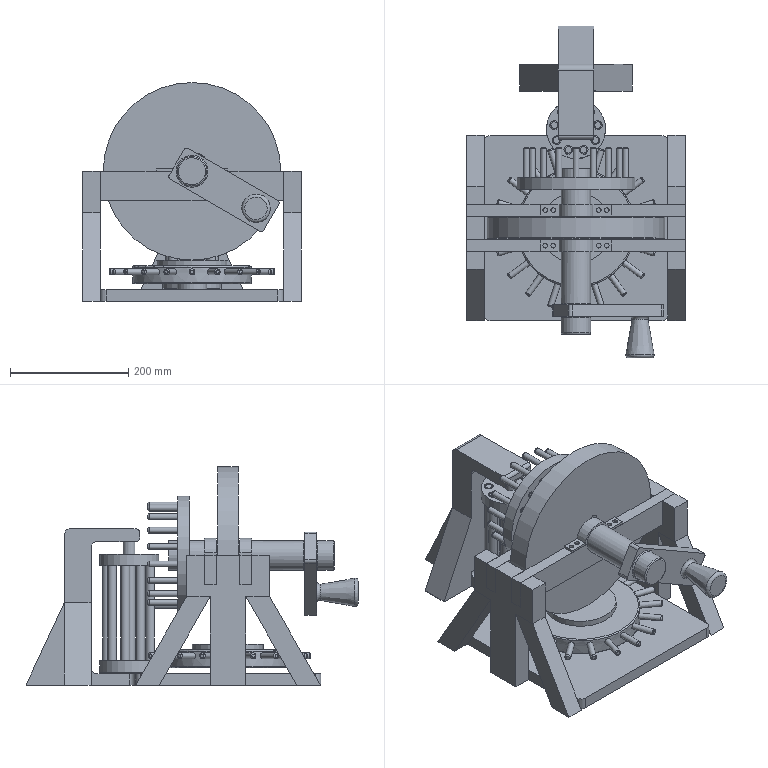Assembly | NX | mm | 67 component files | 67 solids | 525 faces | box 370 x 561.3 x 370 mm | volume 11618898 mm3 | plane 267 | cylinder 154 | torus 103 | cone 1 | commonest cylinder face diameters 10 x80 15 x27 20 x15 50 x10 8 x8 12 x6 200 x2 100 x2
Bill of materials:
unnamed part 1 | 1 |  | Solid obround (stadium-profile) prismatic block: flat parallel faces with fully rounded ends.
unnamed part 2 | 1 |  | Thin flat circular disc with a large central through-hole and a ring of small through-holes evenly spaced around a pitch circle near the outer edge.
unnamed part 3 | 18 |  | Short solid cylindrical pin with small rounded or chamfered edges at both ends.
unnamed part 4 | 1 |  | Bracket: a flat rectangular base plate with rounded corners and one central round hole. A narrow neck tab with a small hole links the plate to a vertical upright. The upright has triangular gussets on both sides and ends in a horizontal hook arm that overhangs back toward the base plate.
unnamed part 5 | 4 |  | Straight rectangular-section bar shaped as an oblique prism: its parallel end faces are cut at an angle instead of square to the length.
unnamed part 6 | 2 |  | Formed strap of constant thickness: a central semicircular arch with a flat flange on each side, each flange having two round through-holes.
unnamed part 7 | 2 |  | Long rectangular-section bar with one semicircular notch through the thickness at the middle of one long edge.
unnamed part 8 | 1 |  | Circular disc or cap with a flat top face, a thick cylindrical rim pierced by a series of radial holes around its circumference, and a smaller central cylindrical boss projecting from the underside.
unnamed part 9 | 20 |  | Slender solid cylindrical rod or pin with small rounded or chamfered edges at both ends.
unnamed part 10 | 9 |  | Very slender solid cylindrical rod with flat ends and slight edge breaks.
unnamed part 11 | 2 |  | Constant-thickness fork- or trident-shaped prismatic block: a rectangular stem topped by a wider crossbar carrying three parallel upright square prongs.
unnamed part 12 | 1 |  | Plain thin solid circular disc with flat parallel faces.
unnamed part 13 | 2 |  | Thick flat circular disc. It has one larger central through-hole and ten smaller through-holes evenly spaced on a circle around it.
unnamed part 14 | 1 |  | Crank-like part made of a flat rectangular arm with rounded corners. A long cylindrical shaft passes through one end of the arm, sticking out a short way on one side and a long way on the other. A tapered, flared knob-like peg sticks out from the other end of the arm on the short-stub side.
unnamed part 15 | 1 |  | Thin flat circular disc with a small central round bore that has a single rectangular notch on one side, consistent with a keyed bore.
unnamed part 16 | 1 |  | Long, slender solid cylindrical rod or pin with plain flat ends that appear slightly chamfered or rounded at the edges.
Mates:
1. touch align | kama 1 face | kol 1 face
2. touch align | kama 1 face | kol 1 face
3. touch align | kol 1 face | tas 1 face
4. touch align | kama 1 face | kol 1 face
5. distance | kama 1 face | kol 1 face
6. distance | kama 1 face | kol 1 face
7. touch align | kama 1 edge | tas 1 face
8. touch align | kama 1 edge | tas 1 face
9. distance | kama 1 face | tas 1 edge
10. touch align | tutucu 2 face | catal 2 face
11. touch align | tutucu 2 face | catal 2 face
12. touch align | tutucu 2 face | catal 2 edge
13. touch align | tutucu 1 face | catal 2 edge
14. touch align | tutucu 1 face | catal 2 face
15. touch align | tutucu 1 face | catal 2 face
16. touch align | ayak 4 edge | catal 2 edge
17. touch align | ayak 4 edge | catal 2 edge
18. touch align | ayak 3 edge | catal 2 edge
19. touch align | ayak 3 edge | catal 2 edge
20. fix | catal 2 component
21. touch align | catal 1 face | tutucu 1 face
22. touch align | tutucu 1 edge | catal 1 edge
23. touch align | tutucu 1 face | catal 1 face
24. fix | catal 1 component
25. touch align | ayak 2 edge | catal 1 edge
26. touch align | ayak 2 edge | catal 1 edge
27. touch align | ayak 1 edge | catal 1 edge
28. touch align | ayak 1 edge | catal 1 edge
29. touch align | ayak 1 edge | catal 1 edge
30. touch align | ayak 1 face | catal 1 face
31. touch align | tutucu 1 face | kol 1 face
32. concentric | cbk2 9 edge | cark1 2 edge
33. concentric | cbk2 9 edge | cark1 1 edge
34. concentric | cbk2 1 edge | cark1 1 edge
35. concentric | cbk2 2 edge | cark1 1 edge
36. concentric | cbk2 3 edge | cark1 1 edge
37. concentric | cbk2 4 edge | cark1 1 edge
38. concentric | cbk2 5 edge | cark1 1 edge
39. concentric | cbk2 6 edge | cark1 1 edge
40. concentric | cbk2 7 edge | cark1 1 edge
41. concentric | cbk2 8 edge | cark1 1 edge
42. concentric | cbk2 1 edge | cark1 2 edge
43. concentric | cbk2 2 edge | cark1 2 edge
44. concentric | cbk2 3 edge | cark1 2 edge
45. concentric | cbk2 4 edge | cark1 2 edge
46. concentric | cbk2 5 edge | cark1 2 edge
47. concentric | cbk2 6 edge | cark1 2 edge
48. concentric | cbk2 7 edge | cark1 2 edge
49. concentric | cbk2 8 edge | cark1 2 edge
50. concentric | cbk2 9 edge | cark1 2 edge
51. concentric | cark3 1 edge | cibik2 18 edge
52. distance | cark1 1 face | kol 1 face
53. concentric | cibik4 20 edge | alt 1 edge
54. fix | assembly component
55. bond | cibik4 20 component | assembly component
56. bond | cibik4 19 component | assembly component
57. bond | cibik4 18 component | assembly component
58. bond | cibik4 17 component | assembly component
59. bond | cibik4 16 component | assembly component
60. bond | cibik4 15 component | assembly component
61. bond | cibik4 14 component | assembly component
62. bond | cibik4 13 component | assembly component
63. bond | cibik4 12 component | assembly component
64. bond | cibik4 11 component | assembly component
65. bond | cibik4 10 component | assembly component
66. bond | cibik4 9 component | assembly component
67. bond | cibik4 8 component | assembly component
68. bond | cibik4 7 component | assembly component
69. bond | cibik4 6 component | assembly component
70. bond | cibik4 5 component | assembly component
71. bond | cibik4 4 component | assembly component
72. bond | cibik4 3 component | assembly component
73. bond | cibik4 2 component | assembly component
74. bond | cibik4 1 component | assembly component
75. circular | assembly datumaxis | assembly cartesiancoordinatesystem | assembly cartesiancoordinatesystem | assembly cartesiancoordinatesystem | assembly cartesiancoordinatesystem | assembly cartesiancoordinatesystem | assembly cartesiancoordinatesystem | assembly cartesiancoordinatesystem | assembly cartesiancoordinatesystem | assembly cartesiancoordinatesystem | assembly cartesiancoordinatesystem | assembly cartesiancoordinatesystem | assembly cartesiancoordinatesystem | assembly cartesiancoordinatesystem | assembly cartesiancoordinatesystem | assembly cartesiancoordinatesystem | assembly cartesiancoordinatesystem | assembly cartesiancoordinatesystem | assembly cartesiancoordinatesystem | assembly cartesiancoordinatesystem | assembly cartesiancoordinatesystem
76. fix | assembly component
77. bond | cibik2 18 component | assembly component
78. bond | cibik2 17 component | assembly component
79. bond | cibik2 16 component | assembly component
80. bond | cibik2 15 component | assembly component
81. bond | cibik2 14 component | assembly component
82. bond | cibik2 13 component | assembly component
83. bond | cibik2 12 component | assembly component
84. bond | cibik2 11 component | assembly component
85. bond | cibik2 10 component | assembly component
86. bond | cibik2 9 component | assembly component
87. bond | cibik2 8 component | assembly component
88. bond | cibik2 7 component | assembly component
89. circular | assembly datumaxis | assembly cartesiancoordinatesystem | assembly cartesiancoordinatesystem | assembly cartesiancoordinatesystem | assembly cartesiancoordinatesystem | assembly cartesiancoordinatesystem | assembly cartesiancoordinatesystem | assembly cartesiancoordinatesystem | assembly cartesiancoordinatesystem | assembly cartesiancoordinatesystem | assembly cartesiancoordinatesystem | assembly cartesiancoordinatesystem | assembly cartesiancoordinatesystem | assembly cartesiancoordinatesystem | assembly cartesiancoordinatesystem | assembly cartesiancoordinatesystem | assembly cartesiancoordinatesystem | assembly cartesiancoordinatesystem | assembly cartesiancoordinatesystem
90. bond | cibik2 6 component | assembly component
91. bond | cibik2 5 component | assembly component
92. bond | cibik2 4 component | assembly component
93. bond | cibik2 3 component | assembly component
94. bond | cibik2 2 component | assembly component
95. bond | cibik2 1 component | assembly component
96. touch align | cam 1 face | alt 1 face
97. touch align | cam 1 face | alt 1 face
98. touch align | kol 1 face | cark3 1 edge
99. distance | ayak 4 face | cibik5 1 face
100. touch align | altlik 1 face | ayak 4 face
101. touch align | altlik 1 face | ayak 3 edge
102. touch align | tuttttucu 1 face | tutucu 2 face
103. touch align | tuttttucu 1 face | tutucu 2 face
104. touch align | tuttttucu 1 edge | tutucu 2 edge
105. fix | tuttttucu 1 component
106. touch align | tuttttucu 2 edge | tutucu 1 edge
107. fix | tuttttucu 2 component